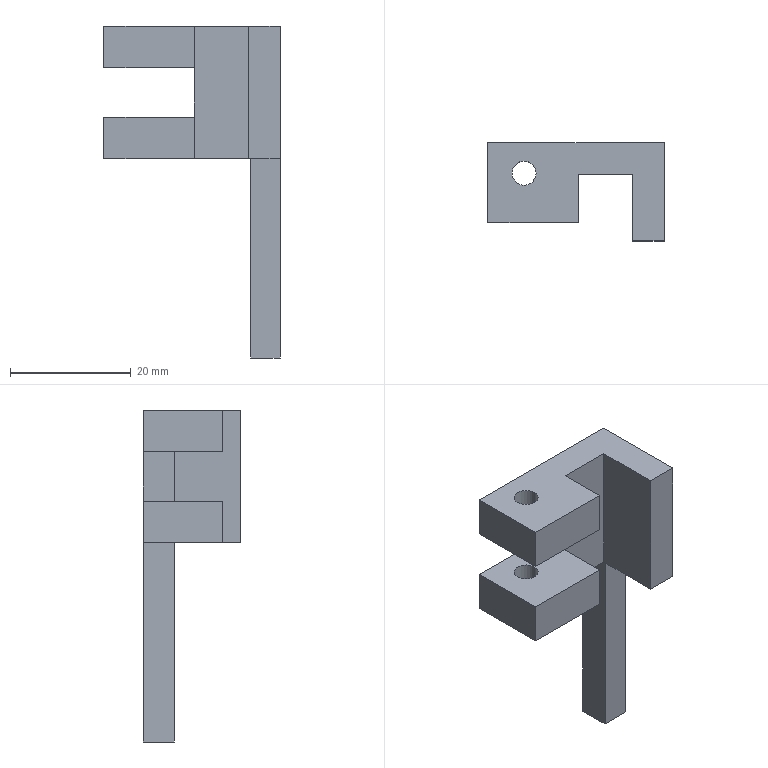Component | SolidWorks | PointedHeadDispensingMovingPart1-1 | 1 solid | 23 faces | box 29.2 x 16.2 x 55 mm | volume 6283 mm3 | plane 19 | cylinder 4 | commonest cylinder face diameters 4 x4
build123d program:
from build123d import *

# Parameters (mm, degrees)
SKETCH1_2_W              = 14.2
SKETCH1_2_H              = 22
EXTRUDE1_DEPTH           = 5.2
SKETCH2_W                = 5.2
SKETCH2_H                = 5.2
EXTRUDE2_DEPTH           = 33
SKETCH3_W                = 22
SKETCH3_H                = 5.2
EXTRUDE3_DEPTH           = 15
SKETCH4_W                = 15
SKETCH4_H                = 22
EXTRUDE4_DEPTH           = 8
SKETCH5_W                = 5.2
SKETCH5_H                = 22
EXTRUDE5_DEPTH           = 11
SKETCH6_W                = 15
SKETCH6_H                = 8.2
CUT_EXTRUDE1_DEPTH       = 59.517
SKETCH7_R                = 2
CUT_EXTRUDE2_DEPTH       = 59.06
SKETCH8_W                = 5.2
SKETCH8_H                = 5.2
CUT_EXTRUDE3_DEPTH       = 33
SKETCH9_W                = 5.2
SKETCH9_H                = 5.2
EXTRUDE6_DEPTH           = 33
PINLANERELIEF_DEPTH      = 38.881
PINLANERELIEF_DEPTH_BACK = 38.881
SKETCH1_W                = 0.3
SKETCH1_H                = 34


with BuildPart() as part:
    # Sketch1_2 → Extrude1 (new body)
    with BuildSketch(Plane(origin=(0, 0, 0), x_dir=(1, 0, 0), z_dir=(0, 1, 0))):
        with Locations((7.1, -11)):
            Rectangle(SKETCH1_2_W, SKETCH1_2_H)
    extrude(amount=EXTRUDE1_DEPTH)

    # Sketch2 → Extrude2 (add)
    with BuildSketch(Plane.XY.offset(22)):
        with Locations((11.6, 2.6)):
            Rectangle(SKETCH2_W, SKETCH2_H)
    extrude(amount=EXTRUDE2_DEPTH)

    # Sketch3 → Extrude3 (add)
    with BuildSketch(Plane.ZY):
        with Locations((11, 2.6)):
            Rectangle(SKETCH3_W, SKETCH3_H)
    extrude(amount=EXTRUDE3_DEPTH)

    # Sketch4 → Extrude4 (add)
    with BuildSketch(Plane.XZ):
        with Locations((-7.5, 11)):
            Rectangle(SKETCH4_W, SKETCH4_H)
    extrude(amount=EXTRUDE4_DEPTH)

    # Sketch5 → Extrude5 (add)
    with BuildSketch(Plane.XZ):
        with Locations((11.6, 11)):
            Rectangle(SKETCH5_W, SKETCH5_H)
    extrude(amount=EXTRUDE5_DEPTH)

    # Sketch6 → Cut-Extrude1 (cut, through all)
    with BuildSketch(Plane.XZ.offset(8)):
        with Locations((-7.5, 11)):
            Rectangle(SKETCH6_W, SKETCH6_H)
    extrude(amount=-CUT_EXTRUDE1_DEPTH, mode=Mode.SUBTRACT)

    # Sketch7 → Cut-Extrude2 (cut, through all)
    with BuildSketch(Plane(origin=(0, 0, 0), x_dir=(-1, 0, 0), z_dir=(0, 0, -1))):
        with Locations((9, 0.2)):
            Circle(SKETCH7_R)
    extrude(amount=-CUT_EXTRUDE2_DEPTH, mode=Mode.SUBTRACT)

    # Sketch8 → Cut-Extrude3 (cut)
    with BuildSketch(Plane.XY.offset(55)):
        with Locations((11.6, 2.6)):
            Rectangle(SKETCH8_W, SKETCH8_H)
    extrude(amount=-CUT_EXTRUDE3_DEPTH, mode=Mode.SUBTRACT)

    # Sketch9 → Extrude6 (add)
    with BuildSketch(Plane(origin=(0, 0, 0), x_dir=(-1, 0, 0), z_dir=(0, 0, -1))):
        with Locations((-11.6, 2.6)):
            Rectangle(SKETCH9_W, SKETCH9_H)
    extrude(amount=EXTRUDE6_DEPTH)

    # Sketch1 → PinLaneRelief (cut, two sides: drawn at the far end of the back side and taken through both)
    with BuildSketch(Plane(origin=(0, 0, 0), x_dir=(1, 0, 0), z_dir=(0, 1, 0)).offset(-PINLANERELIEF_DEPTH_BACK)):
        with Locations((9.15, 17)):
            Rectangle(SKETCH1_W, SKETCH1_H)
    extrude(amount=PINLANERELIEF_DEPTH + PINLANERELIEF_DEPTH_BACK, mode=Mode.SUBTRACT)


solid = part.part

# Placed as in the assembly
solid = solid.moved(Location((10.917, 77.172, -163.887), (0, 0, 0)))
STEP:
#1=COLOUR_RGB('',0.7922,0.8196,0.9333);
#2=FILL_AREA_STYLE_COLOUR('',#1);
#3=FILL_AREA_STYLE('',(#2));
#4=SURFACE_STYLE_FILL_AREA(#3);
#5=SURFACE_SIDE_STYLE('',(#4));
#6=SURFACE_STYLE_USAGE(.BOTH.,#5);
#7=PRESENTATION_STYLE_ASSIGNMENT((#6));
#8=CARTESIAN_POINT('',(0.1542,3.046,-5.586));
#9=VERTEX_POINT('',#8);
#10=CARTESIAN_POINT('',(-0.003273,3.046,-5.586));
#11=VERTEX_POINT('',#10);
#12=CARTESIAN_POINT('',(0.07547,3.046,-5.586));
#13=DIRECTION('',(0.,0.,-1.));
#14=DIRECTION('',(-1.,0.,0.));
#15=AXIS2_PLACEMENT_3D('',#12,#13,#14);
#16=CIRCLE('',#15,0.07874);
#17=EDGE_CURVE('',#9,#11,#16,.T.);
#18=ORIENTED_EDGE('',*,*,#17,.F.);
#19=CARTESIAN_POINT('',(0.1542,3.046,-5.858));
#20=VERTEX_POINT('',#19);
#21=CARTESIAN_POINT('',(0.1542,3.046,-4.287));
#22=DIRECTION('',(0.,0.,-1.));
#23=VECTOR('',#22,39.37);
#24=LINE('',#21,#23);
#25=EDGE_CURVE('',#9,#20,#24,.T.);
#26=ORIENTED_EDGE('',*,*,#25,.T.);
#27=CARTESIAN_POINT('',(-0.003273,3.046,-5.858));
#28=VERTEX_POINT('',#27);
#29=CARTESIAN_POINT('',(0.07547,3.046,-5.858));
#30=DIRECTION('',(0.,0.,1.));
#31=DIRECTION('',(1.,0.,0.));
#32=AXIS2_PLACEMENT_3D('',#29,#30,#31);
#33=CIRCLE('',#32,0.07874);
#34=EDGE_CURVE('',#28,#20,#33,.T.);
#35=ORIENTED_EDGE('',*,*,#34,.F.);
#36=CARTESIAN_POINT('',(-0.003273,3.046,-4.287));
#37=DIRECTION('',(0.,0.,-1.));
#38=VECTOR('',#37,39.37);
#39=LINE('',#36,#38);
#40=EDGE_CURVE('',#11,#28,#39,.T.);
#41=ORIENTED_EDGE('',*,*,#40,.F.);
#42=EDGE_LOOP('',(#18,#26,#35,#41));
#43=FACE_OUTER_BOUND('',#42,.T.);
#44=CARTESIAN_POINT('',(0.07547,3.046,-4.287));
#45=DIRECTION('',(0.,0.,-1.));
#46=DIRECTION('',(-1.,0.,0.));
#47=AXIS2_PLACEMENT_3D('',#44,#45,#46);
#48=CYLINDRICAL_SURFACE('',#47,0.07874);
#49=ADVANCED_FACE('',(#43),#48,.F.);
#50=CARTESIAN_POINT('',(0.1542,3.046,-6.181));
#51=VERTEX_POINT('',#50);
#52=CARTESIAN_POINT('',(-0.003273,3.046,-6.181));
#53=VERTEX_POINT('',#52);
#54=CARTESIAN_POINT('',(0.07547,3.046,-6.181));
#55=DIRECTION('',(0.,0.,-1.));
#56=DIRECTION('',(-1.,0.,0.));
#57=AXIS2_PLACEMENT_3D('',#54,#55,#56);
#58=CIRCLE('',#57,0.07874);
#59=EDGE_CURVE('',#51,#53,#58,.T.);
#60=ORIENTED_EDGE('',*,*,#59,.F.);
#61=CARTESIAN_POINT('',(0.1542,3.046,-6.452));
#62=VERTEX_POINT('',#61);
#63=CARTESIAN_POINT('',(0.1542,3.046,-4.287));
#64=DIRECTION('',(0.,0.,-1.));
#65=VECTOR('',#64,39.37);
#66=LINE('',#63,#65);
#67=EDGE_CURVE('',#51,#62,#66,.T.);
#68=ORIENTED_EDGE('',*,*,#67,.T.);
#69=CARTESIAN_POINT('',(-0.003273,3.046,-6.452));
#70=VERTEX_POINT('',#69);
#71=CARTESIAN_POINT('',(0.07547,3.046,-6.452));
#72=DIRECTION('',(0.,0.,-1.));
#73=DIRECTION('',(-1.,0.,0.));
#74=AXIS2_PLACEMENT_3D('',#71,#72,#73);
#75=CIRCLE('',#74,0.07874);
#76=EDGE_CURVE('',#62,#70,#75,.T.);
#77=ORIENTED_EDGE('',*,*,#76,.T.);
#78=CARTESIAN_POINT('',(-0.003273,3.046,-4.287));
#79=DIRECTION('',(0.,0.,-1.));
#80=VECTOR('',#79,39.37);
#81=LINE('',#78,#80);
#82=EDGE_CURVE('',#53,#70,#81,.T.);
#83=ORIENTED_EDGE('',*,*,#82,.F.);
#84=EDGE_LOOP('',(#60,#68,#77,#83));
#85=FACE_OUTER_BOUND('',#84,.T.);
#86=CARTESIAN_POINT('',(0.07547,3.046,-4.287));
#87=DIRECTION('',(0.,0.,-1.));
#88=DIRECTION('',(-1.,0.,0.));
#89=AXIS2_PLACEMENT_3D('',#86,#87,#88);
#90=CYLINDRICAL_SURFACE('',#89,0.07874);
#91=ADVANCED_FACE('',(#85),#90,.F.);
#92=CARTESIAN_POINT('',(0.9889,3.038,-6.452));
#93=VERTEX_POINT('',#92);
#94=CARTESIAN_POINT('',(0.9889,2.605,-6.452));
#95=VERTEX_POINT('',#94);
#96=CARTESIAN_POINT('',(0.9889,3.243,-6.452));
#97=DIRECTION('',(0.,-1.,0.));
#98=VECTOR('',#97,39.37);
#99=LINE('',#96,#98);
#100=EDGE_CURVE('',#93,#95,#99,.T.);
#101=ORIENTED_EDGE('',*,*,#100,.T.);
#102=CARTESIAN_POINT('',(0.7841,2.605,-6.452));
#103=VERTEX_POINT('',#102);
#104=CARTESIAN_POINT('',(0.7841,2.605,-6.452));
#105=DIRECTION('',(1.,0.,0.));
#106=VECTOR('',#105,39.37);
#107=LINE('',#104,#106);
#108=EDGE_CURVE('',#103,#95,#107,.T.);
#109=ORIENTED_EDGE('',*,*,#108,.F.);
#110=CARTESIAN_POINT('',(0.7841,3.038,-6.452));
#111=VERTEX_POINT('',#110);
#112=CARTESIAN_POINT('',(0.7841,2.605,-6.452));
#113=DIRECTION('',(0.,1.,0.));
#114=VECTOR('',#113,39.37);
#115=LINE('',#112,#114);
#116=EDGE_CURVE('',#103,#111,#115,.T.);
#117=ORIENTED_EDGE('',*,*,#116,.T.);
#118=CARTESIAN_POINT('',(0.4298,3.038,-6.452));
#119=VERTEX_POINT('',#118);
#120=CARTESIAN_POINT('',(0.4298,3.038,-6.452));
#121=DIRECTION('',(-1.,0.,0.));
#122=VECTOR('',#121,39.37);
#123=LINE('',#120,#122);
#124=EDGE_CURVE('',#111,#119,#123,.T.);
#125=ORIENTED_EDGE('',*,*,#124,.T.);
#126=CARTESIAN_POINT('',(0.4298,2.723,-6.452));
#127=VERTEX_POINT('',#126);
#128=CARTESIAN_POINT('',(0.4298,2.723,-6.452));
#129=DIRECTION('',(0.,1.,0.));
#130=VECTOR('',#129,39.37);
#131=LINE('',#128,#130);
#132=EDGE_CURVE('',#127,#119,#131,.T.);
#133=ORIENTED_EDGE('',*,*,#132,.F.);
#134=CARTESIAN_POINT('',(-0.1608,2.723,-6.452));
#135=VERTEX_POINT('',#134);
#136=CARTESIAN_POINT('',(-0.1608,2.723,-6.452));
#137=DIRECTION('',(1.,0.,0.));
#138=VECTOR('',#137,39.37);
#139=LINE('',#136,#138);
#140=EDGE_CURVE('',#135,#127,#139,.T.);
#141=ORIENTED_EDGE('',*,*,#140,.F.);
#142=CARTESIAN_POINT('',(-0.1608,3.243,-6.452));
#143=VERTEX_POINT('',#142);
#144=CARTESIAN_POINT('',(-0.1608,3.243,-6.452));
#145=DIRECTION('',(0.,-1.,0.));
#146=VECTOR('',#145,39.37);
#147=LINE('',#144,#146);
#148=EDGE_CURVE('',#143,#135,#147,.T.);
#149=ORIENTED_EDGE('',*,*,#148,.F.);
#150=CARTESIAN_POINT('',(0.7959,3.243,-6.452));
#151=VERTEX_POINT('',#150);
#152=CARTESIAN_POINT('',(0.4298,3.243,-6.452));
#153=DIRECTION('',(-1.,0.,0.));
#154=VECTOR('',#153,39.37);
#155=LINE('',#152,#154);
#156=EDGE_CURVE('',#151,#143,#155,.T.);
#157=ORIENTED_EDGE('',*,*,#156,.F.);
#158=CARTESIAN_POINT('',(0.7959,3.038,-6.452));
#159=VERTEX_POINT('',#158);
#160=CARTESIAN_POINT('',(0.7959,2.605,-6.452));
#161=DIRECTION('',(0.,1.,0.));
#162=VECTOR('',#161,39.37);
#163=LINE('',#160,#162);
#164=EDGE_CURVE('',#159,#151,#163,.T.);
#165=ORIENTED_EDGE('',*,*,#164,.F.);
#166=CARTESIAN_POINT('',(0.9889,3.038,-6.452));
#167=DIRECTION('',(-1.,0.,0.));
#168=VECTOR('',#167,39.37);
#169=LINE('',#166,#168);
#170=EDGE_CURVE('',#93,#159,#169,.T.);
#171=ORIENTED_EDGE('',*,*,#170,.F.);
#172=EDGE_LOOP('',(#101,#109,#117,#125,#133,#141,#149,#157,#165,#171));
#173=FACE_OUTER_BOUND('',#172,.T.);
#174=CARTESIAN_POINT('',(0.07547,3.046,-6.452));
#175=DIRECTION('',(0.,0.,-1.));
#176=DIRECTION('',(-1.,0.,0.));
#177=AXIS2_PLACEMENT_3D('',#174,#175,#176);
#178=CIRCLE('',#177,0.07874);
#179=EDGE_CURVE('',#70,#62,#178,.T.);
#180=ORIENTED_EDGE('',*,*,#179,.F.);
#181=ORIENTED_EDGE('',*,*,#76,.F.);
#182=EDGE_LOOP('',(#180,#181));
#183=FACE_BOUND('',#182,.T.);
#184=CARTESIAN_POINT('',(0.4298,3.243,-6.452));
#185=DIRECTION('',(0.,0.,1.));
#186=DIRECTION('',(1.,0.,0.));
#187=AXIS2_PLACEMENT_3D('',#184,#185,#186);
#188=PLANE('',#187);
#189=ADVANCED_FACE('',(#173,#183),#188,.F.);
#190=CARTESIAN_POINT('',(-0.1608,3.243,-5.858));
#191=VERTEX_POINT('',#190);
#192=CARTESIAN_POINT('',(-0.1608,2.723,-5.858));
#193=VERTEX_POINT('',#192);
#194=CARTESIAN_POINT('',(-0.1608,3.243,-5.858));
#195=DIRECTION('',(0.,-1.,0.));
#196=VECTOR('',#195,39.37);
#197=LINE('',#194,#196);
#198=EDGE_CURVE('',#191,#193,#197,.T.);
#199=ORIENTED_EDGE('',*,*,#198,.T.);
#200=CARTESIAN_POINT('',(-0.1608,2.723,-5.586));
#201=VERTEX_POINT('',#200);
#202=CARTESIAN_POINT('',(-0.1608,2.723,-5.586));
#203=DIRECTION('',(0.,0.,-1.));
#204=VECTOR('',#203,39.37);
#205=LINE('',#202,#204);
#206=EDGE_CURVE('',#201,#193,#205,.T.);
#207=ORIENTED_EDGE('',*,*,#206,.F.);
#208=CARTESIAN_POINT('',(-0.1608,3.243,-5.586));
#209=VERTEX_POINT('',#208);
#210=CARTESIAN_POINT('',(-0.1608,3.038,-5.586));
#211=DIRECTION('',(0.,1.,0.));
#212=VECTOR('',#211,39.37);
#213=LINE('',#210,#212);
#214=EDGE_CURVE('',#201,#209,#213,.T.);
#215=ORIENTED_EDGE('',*,*,#214,.T.);
#216=CARTESIAN_POINT('',(-0.1608,3.243,-5.586));
#217=DIRECTION('',(-0.,0.,-1.));
#218=VECTOR('',#217,39.37);
#219=LINE('',#216,#218);
#220=EDGE_CURVE('',#209,#191,#219,.T.);
#221=ORIENTED_EDGE('',*,*,#220,.T.);
#222=EDGE_LOOP('',(#199,#207,#215,#221));
#223=FACE_OUTER_BOUND('',#222,.T.);
#224=CARTESIAN_POINT('',(-0.1608,3.038,-6.452));
#225=DIRECTION('',(-1.,0.,0.));
#226=DIRECTION('',(0.,0.,1.));
#227=AXIS2_PLACEMENT_3D('',#224,#225,#226);
#228=PLANE('',#227);
#229=ADVANCED_FACE('',(#223),#228,.T.);
#230=CARTESIAN_POINT('',(0.4298,2.723,-5.858));
#231=VERTEX_POINT('',#230);
#232=CARTESIAN_POINT('',(0.4298,2.723,-5.586));
#233=VERTEX_POINT('',#232);
#234=CARTESIAN_POINT('',(0.4298,2.723,-5.586));
#235=DIRECTION('',(-0.,0.,1.));
#236=VECTOR('',#235,39.37);
#237=LINE('',#234,#236);
#238=EDGE_CURVE('',#231,#233,#237,.T.);
#239=ORIENTED_EDGE('',*,*,#238,.F.);
#240=CARTESIAN_POINT('',(0.4298,3.038,-5.858));
#241=VERTEX_POINT('',#240);
#242=CARTESIAN_POINT('',(0.4298,3.243,-5.858));
#243=DIRECTION('',(0.,-1.,0.));
#244=VECTOR('',#243,39.37);
#245=LINE('',#242,#244);
#246=EDGE_CURVE('',#241,#231,#245,.T.);
#247=ORIENTED_EDGE('',*,*,#246,.F.);
#248=CARTESIAN_POINT('',(0.4298,3.038,-5.586));
#249=VERTEX_POINT('',#248);
#250=CARTESIAN_POINT('',(0.4298,3.038,-5.586));
#251=DIRECTION('',(-0.,0.,1.));
#252=VECTOR('',#251,39.37);
#253=LINE('',#250,#252);
#254=EDGE_CURVE('',#241,#249,#253,.T.);
#255=ORIENTED_EDGE('',*,*,#254,.T.);
#256=CARTESIAN_POINT('',(0.4298,2.723,-5.586));
#257=DIRECTION('',(0.,1.,0.));
#258=VECTOR('',#257,39.37);
#259=LINE('',#256,#258);
#260=EDGE_CURVE('',#233,#249,#259,.T.);
#261=ORIENTED_EDGE('',*,*,#260,.F.);
#262=EDGE_LOOP('',(#239,#247,#255,#261));
#263=FACE_OUTER_BOUND('',#262,.T.);
#264=CARTESIAN_POINT('',(0.4298,2.723,-5.586));
#265=DIRECTION('',(-1.,0.,-0.));
#266=DIRECTION('',(-0.,0.,1.));
#267=AXIS2_PLACEMENT_3D('',#264,#265,#266);
#268=PLANE('',#267);
#269=ADVANCED_FACE('',(#263),#268,.F.);
#270=CARTESIAN_POINT('',(-0.1608,2.723,-5.858));
#271=DIRECTION('',(-1.,0.,0.));
#272=VECTOR('',#271,39.37);
#273=LINE('',#270,#272);
#274=EDGE_CURVE('',#231,#193,#273,.T.);
#275=ORIENTED_EDGE('',*,*,#274,.F.);
#276=ORIENTED_EDGE('',*,*,#238,.T.);
#277=CARTESIAN_POINT('',(-0.1608,2.723,-5.586));
#278=DIRECTION('',(-1.,0.,0.));
#279=VECTOR('',#278,39.37);
#280=LINE('',#277,#279);
#281=EDGE_CURVE('',#233,#201,#280,.T.);
#282=ORIENTED_EDGE('',*,*,#281,.T.);
#283=ORIENTED_EDGE('',*,*,#206,.T.);
#284=EDGE_LOOP('',(#275,#276,#282,#283));
#285=FACE_OUTER_BOUND('',#284,.T.);
#286=CARTESIAN_POINT('',(-0.1608,2.723,-6.452));
#287=DIRECTION('',(0.,-1.,0.));
#288=DIRECTION('',(0.,0.,-1.));
#289=AXIS2_PLACEMENT_3D('',#286,#287,#288);
#290=PLANE('',#289);
#291=ADVANCED_FACE('',(#285),#290,.T.);
#292=CARTESIAN_POINT('',(0.7841,3.038,-5.586));
#293=VERTEX_POINT('',#292);
#294=CARTESIAN_POINT('',(0.7841,3.038,-5.586));
#295=DIRECTION('',(0.,0.,-1.));
#296=VECTOR('',#295,39.37);
#297=LINE('',#294,#296);
#298=EDGE_CURVE('',#293,#111,#297,.T.);
#299=ORIENTED_EDGE('',*,*,#298,.F.);
#300=CARTESIAN_POINT('',(0.4298,3.038,-5.586));
#301=DIRECTION('',(1.,0.,0.));
#302=VECTOR('',#301,39.37);
#303=LINE('',#300,#302);
#304=EDGE_CURVE('',#249,#293,#303,.T.);
#305=ORIENTED_EDGE('',*,*,#304,.F.);
#306=ORIENTED_EDGE('',*,*,#254,.F.);
#307=CARTESIAN_POINT('',(0.4298,3.038,-6.181));
#308=VERTEX_POINT('',#307);
#309=CARTESIAN_POINT('',(0.4298,3.038,-5.586));
#310=DIRECTION('',(0.,0.,-1.));
#311=VECTOR('',#310,39.37);
#312=LINE('',#309,#311);
#313=EDGE_CURVE('',#241,#308,#312,.T.);
#314=ORIENTED_EDGE('',*,*,#313,.T.);
#315=CARTESIAN_POINT('',(0.4298,3.038,-5.586));
#316=DIRECTION('',(-0.,0.,1.));
#317=VECTOR('',#316,39.37);
#318=LINE('',#315,#317);
#319=EDGE_CURVE('',#119,#308,#318,.T.);
#320=ORIENTED_EDGE('',*,*,#319,.F.);
#321=ORIENTED_EDGE('',*,*,#124,.F.);
#322=EDGE_LOOP('',(#299,#305,#306,#314,#320,#321));
#323=FACE_OUTER_BOUND('',#322,.T.);
#324=CARTESIAN_POINT('',(0.4298,3.038,-5.586));
#325=DIRECTION('',(0.,1.,0.));
#326=DIRECTION('',(0.,0.,1.));
#327=AXIS2_PLACEMENT_3D('',#324,#325,#326);
#328=PLANE('',#327);
#329=ADVANCED_FACE('',(#323),#328,.F.);
#330=CARTESIAN_POINT('',(0.07547,3.046,-5.586));
#331=DIRECTION('',(0.,0.,-1.));
#332=DIRECTION('',(-1.,0.,0.));
#333=AXIS2_PLACEMENT_3D('',#330,#331,#332);
#334=CIRCLE('',#333,0.07874);
#335=EDGE_CURVE('',#11,#9,#334,.T.);
#336=ORIENTED_EDGE('',*,*,#335,.T.);
#337=ORIENTED_EDGE('',*,*,#17,.T.);
#338=EDGE_LOOP('',(#336,#337));
#339=FACE_BOUND('',#338,.T.);
#340=ORIENTED_EDGE('',*,*,#304,.T.);
#341=CARTESIAN_POINT('',(0.7841,2.605,-5.586));
#342=VERTEX_POINT('',#341);
#343=CARTESIAN_POINT('',(0.7841,2.605,-5.586));
#344=DIRECTION('',(0.,1.,0.));
#345=VECTOR('',#344,39.37);
#346=LINE('',#343,#345);
#347=EDGE_CURVE('',#342,#293,#346,.T.);
#348=ORIENTED_EDGE('',*,*,#347,.F.);
#349=CARTESIAN_POINT('',(0.9889,2.605,-5.586));
#350=VERTEX_POINT('',#349);
#351=CARTESIAN_POINT('',(0.7841,2.605,-5.586));
#352=DIRECTION('',(-1.,0.,0.));
#353=VECTOR('',#352,39.37);
#354=LINE('',#351,#353);
#355=EDGE_CURVE('',#350,#342,#354,.T.);
#356=ORIENTED_EDGE('',*,*,#355,.F.);
#357=CARTESIAN_POINT('',(0.9889,3.243,-5.586));
#358=VERTEX_POINT('',#357);
#359=CARTESIAN_POINT('',(0.9889,2.605,-5.586));
#360=DIRECTION('',(0.,1.,0.));
#361=VECTOR('',#360,39.37);
#362=LINE('',#359,#361);
#363=EDGE_CURVE('',#350,#358,#362,.T.);
#364=ORIENTED_EDGE('',*,*,#363,.T.);
#365=CARTESIAN_POINT('',(0.4298,3.243,-5.586));
#366=DIRECTION('',(1.,0.,0.));
#367=VECTOR('',#366,39.37);
#368=LINE('',#365,#367);
#369=EDGE_CURVE('',#209,#358,#368,.T.);
#370=ORIENTED_EDGE('',*,*,#369,.F.);
#371=ORIENTED_EDGE('',*,*,#214,.F.);
#372=ORIENTED_EDGE('',*,*,#281,.F.);
#373=ORIENTED_EDGE('',*,*,#260,.T.);
#374=EDGE_LOOP('',(#340,#348,#356,#364,#370,#371,#372,#373));
#375=FACE_OUTER_BOUND('',#374,.T.);
#376=CARTESIAN_POINT('',(0.4298,3.243,-5.586));
#377=DIRECTION('',(0.,0.,-1.));
#378=DIRECTION('',(-1.,0.,0.));
#379=AXIS2_PLACEMENT_3D('',#376,#377,#378);
#380=PLANE('',#379);
#381=ADVANCED_FACE('',(#339,#375),#380,.F.);
#382=CARTESIAN_POINT('',(0.9889,3.243,-7.751));
#383=VERTEX_POINT('',#382);
#384=CARTESIAN_POINT('',(0.9889,3.243,-6.452));
#385=DIRECTION('',(-0.,0.,-1.));
#386=VECTOR('',#385,39.37);
#387=LINE('',#384,#386);
#388=EDGE_CURVE('',#358,#383,#387,.T.);
#389=ORIENTED_EDGE('',*,*,#388,.F.);
#390=ORIENTED_EDGE('',*,*,#363,.F.);
#391=CARTESIAN_POINT('',(0.9889,2.605,-5.586));
#392=DIRECTION('',(-0.,0.,1.));
#393=VECTOR('',#392,39.37);
#394=LINE('',#391,#393);
#395=EDGE_CURVE('',#95,#350,#394,.T.);
#396=ORIENTED_EDGE('',*,*,#395,.F.);
#397=ORIENTED_EDGE('',*,*,#100,.F.);
#398=CARTESIAN_POINT('',(0.9889,3.038,-7.751));
#399=VERTEX_POINT('',#398);
#400=CARTESIAN_POINT('',(0.9889,3.038,-7.751));
#401=DIRECTION('',(0.,0.,1.));
#402=VECTOR('',#401,39.37);
#403=LINE('',#400,#402);
#404=EDGE_CURVE('',#399,#93,#403,.T.);
#405=ORIENTED_EDGE('',*,*,#404,.F.);
#406=CARTESIAN_POINT('',(0.9889,3.243,-7.751));
#407=DIRECTION('',(0.,-1.,0.));
#408=VECTOR('',#407,39.37);
#409=LINE('',#406,#408);
#410=EDGE_CURVE('',#383,#399,#409,.T.);
#411=ORIENTED_EDGE('',*,*,#410,.F.);
#412=EDGE_LOOP('',(#389,#390,#396,#397,#405,#411));
#413=FACE_OUTER_BOUND('',#412,.T.);
#414=CARTESIAN_POINT('',(0.9889,3.243,-6.452));
#415=DIRECTION('',(-1.,0.,0.));
#416=DIRECTION('',(0.,0.,1.));
#417=AXIS2_PLACEMENT_3D('',#414,#415,#416);
#418=PLANE('',#417);
#419=ADVANCED_FACE('',(#413),#418,.F.);
#420=CARTESIAN_POINT('',(0.7959,3.243,-7.751));
#421=VERTEX_POINT('',#420);
#422=CARTESIAN_POINT('',(0.7959,3.243,-5.586));
#423=DIRECTION('',(0.,0.,-1.));
#424=VECTOR('',#423,39.37);
#425=LINE('',#422,#424);
#426=EDGE_CURVE('',#151,#421,#425,.T.);
#427=ORIENTED_EDGE('',*,*,#426,.F.);
#428=ORIENTED_EDGE('',*,*,#156,.T.);
#429=CARTESIAN_POINT('',(-0.1608,3.243,-6.181));
#430=VERTEX_POINT('',#429);
#431=CARTESIAN_POINT('',(-0.1608,3.243,-5.586));
#432=DIRECTION('',(-0.,0.,-1.));
#433=VECTOR('',#432,39.37);
#434=LINE('',#431,#433);
#435=EDGE_CURVE('',#430,#143,#434,.T.);
#436=ORIENTED_EDGE('',*,*,#435,.F.);
#437=CARTESIAN_POINT('',(0.4298,3.243,-6.181));
#438=VERTEX_POINT('',#437);
#439=CARTESIAN_POINT('',(0.4298,3.243,-6.181));
#440=DIRECTION('',(-1.,0.,0.));
#441=VECTOR('',#440,39.37);
#442=LINE('',#439,#441);
#443=EDGE_CURVE('',#438,#430,#442,.T.);
#444=ORIENTED_EDGE('',*,*,#443,.F.);
#445=CARTESIAN_POINT('',(0.4298,3.243,-5.858));
#446=VERTEX_POINT('',#445);
#447=CARTESIAN_POINT('',(0.4298,3.243,-5.586));
#448=DIRECTION('',(0.,0.,-1.));
#449=VECTOR('',#448,39.37);
#450=LINE('',#447,#449);
#451=EDGE_CURVE('',#446,#438,#450,.T.);
#452=ORIENTED_EDGE('',*,*,#451,.F.);
#453=CARTESIAN_POINT('',(0.4298,3.243,-5.858));
#454=DIRECTION('',(1.,0.,0.));
#455=VECTOR('',#454,39.37);
#456=LINE('',#453,#455);
#457=EDGE_CURVE('',#191,#446,#456,.T.);
#458=ORIENTED_EDGE('',*,*,#457,.F.);
#459=ORIENTED_EDGE('',*,*,#220,.F.);
#460=ORIENTED_EDGE('',*,*,#369,.T.);
#461=ORIENTED_EDGE('',*,*,#388,.T.);
#462=CARTESIAN_POINT('',(0.9889,3.243,-7.751));
#463=DIRECTION('',(1.,0.,0.));
#464=VECTOR('',#463,39.37);
#465=LINE('',#462,#464);
#466=EDGE_CURVE('',#421,#383,#465,.T.);
#467=ORIENTED_EDGE('',*,*,#466,.F.);
#468=EDGE_LOOP('',(#427,#428,#436,#444,#452,#458,#459,#460,#461,#467));
#469=FACE_OUTER_BOUND('',#468,.T.);
#470=CARTESIAN_POINT('',(0.4298,3.243,-5.586));
#471=DIRECTION('',(0.,1.,0.));
#472=DIRECTION('',(0.,0.,1.));
#473=AXIS2_PLACEMENT_3D('',#470,#471,#472);
#474=PLANE('',#473);
#475=ADVANCED_FACE('',(#469),#474,.T.);
#476=CARTESIAN_POINT('',(-0.1608,2.723,-6.181));
#477=VERTEX_POINT('',#476);
#478=CARTESIAN_POINT('',(-0.1608,3.243,-6.181));
#479=DIRECTION('',(0.,-1.,0.));
#480=VECTOR('',#479,39.37);
#481=LINE('',#478,#480);
#482=EDGE_CURVE('',#430,#477,#481,.T.);
#483=ORIENTED_EDGE('',*,*,#482,.F.);
#484=ORIENTED_EDGE('',*,*,#435,.T.);
#485=ORIENTED_EDGE('',*,*,#148,.T.);
#486=CARTESIAN_POINT('',(-0.1608,2.723,-5.586));
#487=DIRECTION('',(0.,0.,-1.));
#488=VECTOR('',#487,39.37);
#489=LINE('',#486,#488);
#490=EDGE_CURVE('',#477,#135,#489,.T.);
#491=ORIENTED_EDGE('',*,*,#490,.F.);
#492=EDGE_LOOP('',(#483,#484,#485,#491));
#493=FACE_OUTER_BOUND('',#492,.T.);
#494=CARTESIAN_POINT('',(-0.1608,3.038,-6.452));
#495=DIRECTION('',(-1.,0.,0.));
#496=DIRECTION('',(0.,0.,1.));
#497=AXIS2_PLACEMENT_3D('',#494,#495,#496);
#498=PLANE('',#497);
#499=ADVANCED_FACE('',(#493),#498,.T.);
#500=ORIENTED_EDGE('',*,*,#319,.T.);
#501=CARTESIAN_POINT('',(0.4298,2.723,-6.181));
#502=VERTEX_POINT('',#501);
#503=CARTESIAN_POINT('',(0.4298,3.243,-6.181));
#504=DIRECTION('',(0.,-1.,0.));
#505=VECTOR('',#504,39.37);
#506=LINE('',#503,#505);
#507=EDGE_CURVE('',#308,#502,#506,.T.);
#508=ORIENTED_EDGE('',*,*,#507,.T.);
#509=CARTESIAN_POINT('',(0.4298,2.723,-5.586));
#510=DIRECTION('',(-0.,0.,1.));
#511=VECTOR('',#510,39.37);
#512=LINE('',#509,#511);
#513=EDGE_CURVE('',#127,#502,#512,.T.);
#514=ORIENTED_EDGE('',*,*,#513,.F.);
#515=ORIENTED_EDGE('',*,*,#132,.T.);
#516=EDGE_LOOP('',(#500,#508,#514,#515));
#517=FACE_OUTER_BOUND('',#516,.T.);
#518=CARTESIAN_POINT('',(0.4298,2.723,-5.586));
#519=DIRECTION('',(-1.,0.,-0.));
#520=DIRECTION('',(-0.,0.,1.));
#521=AXIS2_PLACEMENT_3D('',#518,#519,#520);
#522=PLANE('',#521);
#523=ADVANCED_FACE('',(#517),#522,.F.);
#524=CARTESIAN_POINT('',(-0.1608,2.723,-6.181));
#525=DIRECTION('',(1.,0.,0.));
#526=VECTOR('',#525,39.37);
#527=LINE('',#524,#526);
#528=EDGE_CURVE('',#477,#502,#527,.T.);
#529=ORIENTED_EDGE('',*,*,#528,.F.);
#530=ORIENTED_EDGE('',*,*,#490,.T.);
#531=ORIENTED_EDGE('',*,*,#140,.T.);
#532=ORIENTED_EDGE('',*,*,#513,.T.);
#533=EDGE_LOOP('',(#529,#530,#531,#532));
#534=FACE_OUTER_BOUND('',#533,.T.);
#535=CARTESIAN_POINT('',(-0.1608,2.723,-6.452));
#536=DIRECTION('',(0.,-1.,0.));
#537=DIRECTION('',(0.,0.,-1.));
#538=AXIS2_PLACEMENT_3D('',#535,#536,#537);
#539=PLANE('',#538);
#540=ADVANCED_FACE('',(#534),#539,.T.);
#541=ORIENTED_EDGE('',*,*,#298,.T.);
#542=ORIENTED_EDGE('',*,*,#116,.F.);
#543=CARTESIAN_POINT('',(0.7841,2.605,-5.586));
#544=DIRECTION('',(0.,0.,-1.));
#545=VECTOR('',#544,39.37);
#546=LINE('',#543,#545);
#547=EDGE_CURVE('',#342,#103,#546,.T.);
#548=ORIENTED_EDGE('',*,*,#547,.F.);
#549=ORIENTED_EDGE('',*,*,#347,.T.);
#550=EDGE_LOOP('',(#541,#542,#548,#549));
#551=FACE_OUTER_BOUND('',#550,.T.);
#552=CARTESIAN_POINT('',(0.7841,2.605,-5.586));
#553=DIRECTION('',(1.,0.,0.));
#554=DIRECTION('',(0.,0.,-1.));
#555=AXIS2_PLACEMENT_3D('',#552,#553,#554);
#556=PLANE('',#555);
#557=ADVANCED_FACE('',(#551),#556,.F.);
#558=ORIENTED_EDGE('',*,*,#547,.T.);
#559=ORIENTED_EDGE('',*,*,#108,.T.);
#560=ORIENTED_EDGE('',*,*,#395,.T.);
#561=ORIENTED_EDGE('',*,*,#355,.T.);
#562=EDGE_LOOP('',(#558,#559,#560,#561));
#563=FACE_OUTER_BOUND('',#562,.T.);
#564=CARTESIAN_POINT('',(0.7841,2.605,-6.452));
#565=DIRECTION('',(0.,-1.,0.));
#566=DIRECTION('',(0.,0.,-1.));
#567=AXIS2_PLACEMENT_3D('',#564,#565,#566);
#568=PLANE('',#567);
#569=ADVANCED_FACE('',(#563),#568,.T.);
#570=CARTESIAN_POINT('',(0.4298,3.243,-5.858));
#571=DIRECTION('',(0.,-1.,0.));
#572=VECTOR('',#571,39.37);
#573=LINE('',#570,#572);
#574=EDGE_CURVE('',#446,#241,#573,.T.);
#575=ORIENTED_EDGE('',*,*,#574,.F.);
#576=ORIENTED_EDGE('',*,*,#451,.T.);
#577=CARTESIAN_POINT('',(0.4298,3.243,-6.181));
#578=DIRECTION('',(0.,-1.,0.));
#579=VECTOR('',#578,39.37);
#580=LINE('',#577,#579);
#581=EDGE_CURVE('',#438,#308,#580,.T.);
#582=ORIENTED_EDGE('',*,*,#581,.T.);
#583=ORIENTED_EDGE('',*,*,#313,.F.);
#584=EDGE_LOOP('',(#575,#576,#582,#583));
#585=FACE_OUTER_BOUND('',#584,.T.);
#586=CARTESIAN_POINT('',(0.4298,3.243,-5.858));
#587=DIRECTION('',(1.,0.,0.));
#588=DIRECTION('',(0.,0.,-1.));
#589=AXIS2_PLACEMENT_3D('',#586,#587,#588);
#590=PLANE('',#589);
#591=ADVANCED_FACE('',(#585),#590,.F.);
#592=ORIENTED_EDGE('',*,*,#34,.T.);
#593=CARTESIAN_POINT('',(0.07547,3.046,-5.858));
#594=DIRECTION('',(0.,0.,1.));
#595=DIRECTION('',(1.,0.,0.));
#596=AXIS2_PLACEMENT_3D('',#593,#594,#595);
#597=CIRCLE('',#596,0.07874);
#598=EDGE_CURVE('',#20,#28,#597,.T.);
#599=ORIENTED_EDGE('',*,*,#598,.T.);
#600=EDGE_LOOP('',(#592,#599));
#601=FACE_BOUND('',#600,.T.);
#602=ORIENTED_EDGE('',*,*,#457,.T.);
#603=ORIENTED_EDGE('',*,*,#574,.T.);
#604=ORIENTED_EDGE('',*,*,#246,.T.);
#605=ORIENTED_EDGE('',*,*,#274,.T.);
#606=ORIENTED_EDGE('',*,*,#198,.F.);
#607=EDGE_LOOP('',(#602,#603,#604,#605,#606));
#608=FACE_OUTER_BOUND('',#607,.T.);
#609=CARTESIAN_POINT('',(-0.1608,3.243,-5.858));
#610=DIRECTION('',(0.,0.,1.));
#611=DIRECTION('',(1.,0.,0.));
#612=AXIS2_PLACEMENT_3D('',#609,#610,#611);
#613=PLANE('',#612);
#614=ADVANCED_FACE('',(#601,#608),#613,.F.);
#615=CARTESIAN_POINT('',(0.07547,3.046,-6.181));
#616=DIRECTION('',(0.,0.,-1.));
#617=DIRECTION('',(-1.,0.,0.));
#618=AXIS2_PLACEMENT_3D('',#615,#616,#617);
#619=CIRCLE('',#618,0.07874);
#620=EDGE_CURVE('',#53,#51,#619,.T.);
#621=ORIENTED_EDGE('',*,*,#620,.T.);
#622=ORIENTED_EDGE('',*,*,#59,.T.);
#623=EDGE_LOOP('',(#621,#622));
#624=FACE_BOUND('',#623,.T.);
#625=ORIENTED_EDGE('',*,*,#443,.T.);
#626=ORIENTED_EDGE('',*,*,#482,.T.);
#627=ORIENTED_EDGE('',*,*,#528,.T.);
#628=ORIENTED_EDGE('',*,*,#507,.F.);
#629=ORIENTED_EDGE('',*,*,#581,.F.);
#630=EDGE_LOOP('',(#625,#626,#627,#628,#629));
#631=FACE_OUTER_BOUND('',#630,.T.);
#632=CARTESIAN_POINT('',(-0.1608,3.243,-6.181));
#633=DIRECTION('',(0.,0.,-1.));
#634=DIRECTION('',(-1.,0.,0.));
#635=AXIS2_PLACEMENT_3D('',#632,#633,#634);
#636=PLANE('',#635);
#637=ADVANCED_FACE('',(#624,#631),#636,.F.);
#638=ORIENTED_EDGE('',*,*,#67,.F.);
#639=ORIENTED_EDGE('',*,*,#620,.F.);
#640=ORIENTED_EDGE('',*,*,#82,.T.);
#641=ORIENTED_EDGE('',*,*,#179,.T.);
#642=EDGE_LOOP('',(#638,#639,#640,#641));
#643=FACE_OUTER_BOUND('',#642,.T.);
#644=CARTESIAN_POINT('',(0.07547,3.046,-4.287));
#645=DIRECTION('',(0.,0.,-1.));
#646=DIRECTION('',(-1.,0.,0.));
#647=AXIS2_PLACEMENT_3D('',#644,#645,#646);
#648=CYLINDRICAL_SURFACE('',#647,0.07874);
#649=ADVANCED_FACE('',(#643),#648,.F.);
#650=ORIENTED_EDGE('',*,*,#25,.F.);
#651=ORIENTED_EDGE('',*,*,#335,.F.);
#652=ORIENTED_EDGE('',*,*,#40,.T.);
#653=ORIENTED_EDGE('',*,*,#598,.F.);
#654=EDGE_LOOP('',(#650,#651,#652,#653));
#655=FACE_OUTER_BOUND('',#654,.T.);
#656=CARTESIAN_POINT('',(0.07547,3.046,-4.287));
#657=DIRECTION('',(0.,0.,-1.));
#658=DIRECTION('',(-1.,0.,0.));
#659=AXIS2_PLACEMENT_3D('',#656,#657,#658);
#660=CYLINDRICAL_SURFACE('',#659,0.07874);
#661=ADVANCED_FACE('',(#655),#660,.F.);
#662=ORIENTED_EDGE('',*,*,#170,.T.);
#663=CARTESIAN_POINT('',(0.7959,3.038,-7.751));
#664=VERTEX_POINT('',#663);
#665=CARTESIAN_POINT('',(0.7959,3.038,-7.751));
#666=DIRECTION('',(0.,0.,-1.));
#667=VECTOR('',#666,39.37);
#668=LINE('',#665,#667);
#669=EDGE_CURVE('',#159,#664,#668,.T.);
#670=ORIENTED_EDGE('',*,*,#669,.T.);
#671=CARTESIAN_POINT('',(0.9889,3.038,-7.751));
#672=DIRECTION('',(-1.,0.,0.));
#673=VECTOR('',#672,39.37);
#674=LINE('',#671,#673);
#675=EDGE_CURVE('',#399,#664,#674,.T.);
#676=ORIENTED_EDGE('',*,*,#675,.F.);
#677=ORIENTED_EDGE('',*,*,#404,.T.);
#678=EDGE_LOOP('',(#662,#670,#676,#677));
#679=FACE_OUTER_BOUND('',#678,.T.);
#680=CARTESIAN_POINT('',(0.9889,3.038,-7.751));
#681=DIRECTION('',(0.,1.,0.));
#682=DIRECTION('',(0.,0.,1.));
#683=AXIS2_PLACEMENT_3D('',#680,#681,#682);
#684=PLANE('',#683);
#685=ADVANCED_FACE('',(#679),#684,.F.);
#686=CARTESIAN_POINT('',(0.7959,3.038,-7.751));
#687=DIRECTION('',(0.,-1.,0.));
#688=VECTOR('',#687,39.37);
#689=LINE('',#686,#688);
#690=EDGE_CURVE('',#421,#664,#689,.T.);
#691=ORIENTED_EDGE('',*,*,#690,.F.);
#692=ORIENTED_EDGE('',*,*,#466,.T.);
#693=ORIENTED_EDGE('',*,*,#410,.T.);
#694=ORIENTED_EDGE('',*,*,#675,.T.);
#695=EDGE_LOOP('',(#691,#692,#693,#694));
#696=FACE_OUTER_BOUND('',#695,.T.);
#697=CARTESIAN_POINT('',(0.9889,3.038,-7.751));
#698=DIRECTION('',(0.,0.,-1.));
#699=DIRECTION('',(-1.,0.,0.));
#700=AXIS2_PLACEMENT_3D('',#697,#698,#699);
#701=PLANE('',#700);
#702=ADVANCED_FACE('',(#696),#701,.T.);
#703=ORIENTED_EDGE('',*,*,#164,.T.);
#704=ORIENTED_EDGE('',*,*,#426,.T.);
#705=ORIENTED_EDGE('',*,*,#690,.T.);
#706=ORIENTED_EDGE('',*,*,#669,.F.);
#707=EDGE_LOOP('',(#703,#704,#705,#706));
#708=FACE_OUTER_BOUND('',#707,.T.);
#709=CARTESIAN_POINT('',(0.7959,2.605,-7.791));
#710=DIRECTION('',(1.,0.,0.));
#711=DIRECTION('',(0.,0.,-1.));
#712=AXIS2_PLACEMENT_3D('',#709,#710,#711);
#713=PLANE('',#712);
#714=ADVANCED_FACE('',(#708),#713,.F.);
#715=CLOSED_SHELL('',(#49,#91,#189,#229,#269,#291,#329,#381,#419,#475,#499,#523,#540,#557,#569,#591,#614,#637,#649,#661,#685,#702,#714));
#716=MANIFOLD_SOLID_BREP('',#715);
#717=STYLED_ITEM('',(#7),#716);
#718=PRESENTATION_LAYER_ASSIGNMENT('','',(#717));
#719=CARTESIAN_POINT('',(0.,0.,0.));
#720=DIRECTION('',(0.,0.,1.));
#721=DIRECTION('',(1.,0.,0.));
#722=AXIS2_PLACEMENT_3D('',#719,#720,#721);
#723=(LENGTH_UNIT()NAMED_UNIT(*)SI_UNIT($,.METRE.));
#724=LENGTH_MEASURE_WITH_UNIT(LENGTH_MEASURE(0.0254),#723);
#725=DIMENSIONAL_EXPONENTS(1.,0.,0.,0.,0.,0.,0.);
#726=(CONVERSION_BASED_UNIT('',#724)LENGTH_UNIT()NAMED_UNIT(#725));
#727=UNCERTAINTY_MEASURE_WITH_UNIT(LENGTH_MEASURE(0.00001),#726,'','');
#728=(NAMED_UNIT(*)PLANE_ANGLE_UNIT()SI_UNIT($,.RADIAN.));
#729=(NAMED_UNIT(*)SI_UNIT($,.STERADIAN.)SOLID_ANGLE_UNIT());
#730=(GEOMETRIC_REPRESENTATION_CONTEXT(3)GLOBAL_UNCERTAINTY_ASSIGNED_CONTEXT((#727))GLOBAL_UNIT_ASSIGNED_CONTEXT((#726,#728,#729))REPRESENTATION_CONTEXT('',''));
#731=ADVANCED_BREP_SHAPE_REPRESENTATION('',(#716,#722),#730);
#732=(LENGTH_UNIT()NAMED_UNIT(*)SI_UNIT($,.METRE.));
#733=LENGTH_MEASURE_WITH_UNIT(LENGTH_MEASURE(0.0254),#732);
#734=DIMENSIONAL_EXPONENTS(1.,0.,0.,0.,0.,0.,0.);
#735=(CONVERSION_BASED_UNIT('',#733)LENGTH_UNIT()NAMED_UNIT(#734));
#736=UNCERTAINTY_MEASURE_WITH_UNIT(LENGTH_MEASURE(0.00001),#735,'','');
#737=(NAMED_UNIT(*)PLANE_ANGLE_UNIT()SI_UNIT($,.RADIAN.));
#738=(NAMED_UNIT(*)SI_UNIT($,.STERADIAN.)SOLID_ANGLE_UNIT());
#739=(GEOMETRIC_REPRESENTATION_CONTEXT(3)GLOBAL_UNCERTAINTY_ASSIGNED_CONTEXT((#736))GLOBAL_UNIT_ASSIGNED_CONTEXT((#735,#737,#738))REPRESENTATION_CONTEXT('',''));
#740=MECHANICAL_DESIGN_GEOMETRIC_PRESENTATION_REPRESENTATION('',(#717),#739);